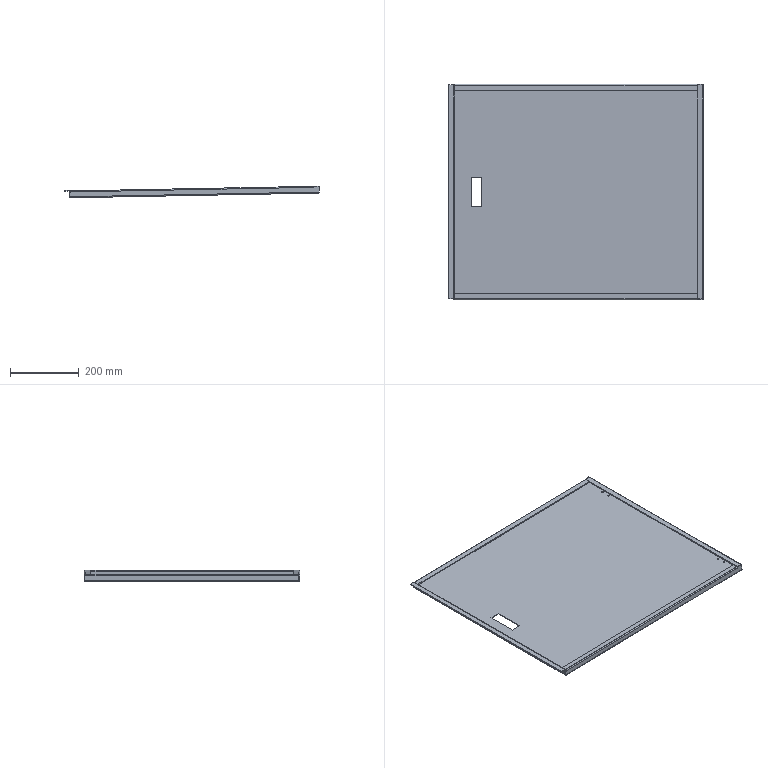Component | SolidWorks | 23BottomDoor2-2 | 1 solid | 98 faces | volume 1077611 mm3 | plane 74 | cylinder 24 | commonest cylinder face diameters 4.2 x8 6 x8 2 x8 | material A3 Steel